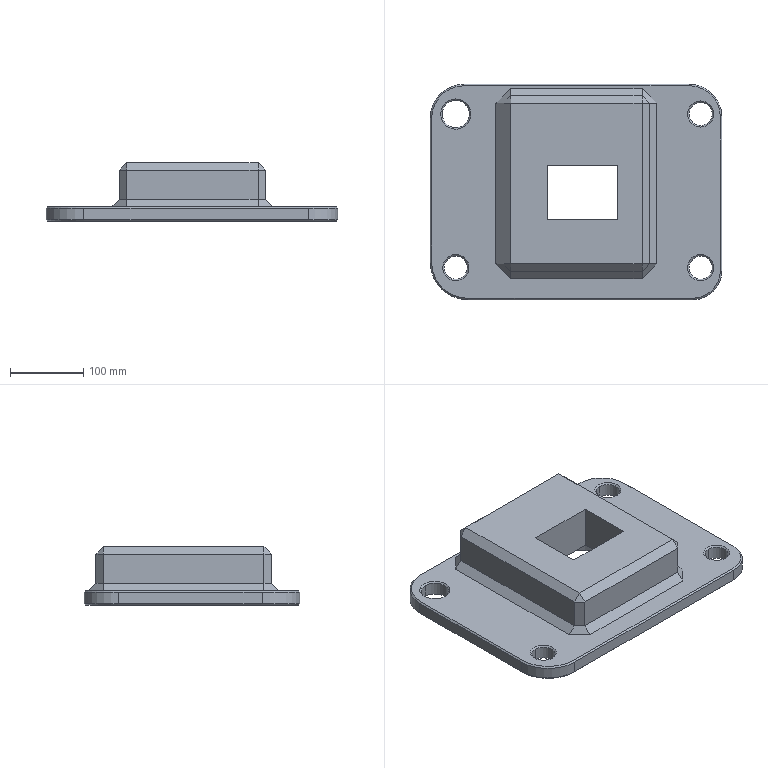Component | SolidWorks | PressurePlate-1 | 1 solid | 74 faces | box 399.22 x 295 x 80 mm | volume 4340570 mm3 | plane 44 | cone 16 | cylinder 14 | commonest cylinder face diameters 31.719 x6 37.423 x2 148.471 x2 79.887 x1 89.44 x1 93.338 x1 103.082 x1
build123d program:
from build123d import *

# Parameters (mm, degrees)
SKETCH1_W             = 295
SKETCH1_H             = 399.223
BOSS_EXTRUDE1_DEPTH   = 20
SKETCH2_W             = 240
SKETCH2_H             = 200
BOSS_EXTRUDE2_DEPTH   = 60
SKETCH3_W             = 74
SKETCH3_H             = 96
CUT_EXTRUDE1_DEPTH    = 267.314
SKETCH4_W             = 74.236
SKETCH4_H             = 20
M27_CLEARANCE_HOLE1_D = 31.719
M33_CLEARANCE_HOLE1_D = 37.423
CHAMFER1_SIZE         = 10
FILLET1_R             = 39.943
FILLET2_R             = 44.72
FILLET3_R             = 46.669
FILLET4_R             = 51.541
CHAMFER2_SIZE2        = 2
CHAMFER2_SIZE         = 2


with BuildPart() as part:
    # Sketch1 → Boss-Extrude1 (new body)
    with BuildSketch(Plane(origin=(0, 0, 190), x_dir=(-1, 0, 0), z_dir=(0, 0, -1))):
        with Locations((-0.5549, -6.793)):
            Rectangle(SKETCH1_W, SKETCH1_H)
    extrude(amount=-BOSS_EXTRUDE1_DEPTH)

    # Sketch2 → Boss-Extrude2 (add)
    with BuildSketch(Plane(origin=(0, 0, 190), x_dir=(-1, 0, 0), z_dir=(0, 0, -1))):
        with Locations((-12.055, -6.405)):
            Rectangle(SKETCH2_W, SKETCH2_H)
    extrude(amount=BOSS_EXTRUDE2_DEPTH)

    # Sketch3 → Cut-Extrude1 (cut, through all)
    with BuildSketch(Plane.XY.offset(210)):
        with Locations((0.05486, 1.595)):
            Rectangle(SKETCH3_W, SKETCH3_H)
    extrude(amount=-CUT_EXTRUDE1_DEPTH, mode=Mode.SUBTRACT)

    # Sketch4 → Cut-Revolve1 (revolve, cut)
    with BuildSketch(Plane(origin=(0, 2.202, 0), x_dir=(1, 0, 0), z_dir=(0, 1, 0))):
        with Locations((-34.987, -200)):
            Rectangle(SKETCH4_W, SKETCH4_H)
    revolve(axis=Axis((2.131, 2.202, 210), (0, 0, -1)), mode=Mode.SUBTRACT)

    # M27 Clearance Hole1 (through all)
    with Locations(Plane(origin=(0, 0, 190), x_dir=(-1, 0, 0), z_dir=(0, 0, -1))):
        with Locations((102.968, -171.325), (102.968, 163.809), (-107.267, 163.809)):
            Hole(M27_CLEARANCE_HOLE1_D / 2)

    # M33 Clearance Hole1 (through all)
    with Locations(Plane(origin=(0, 0, 190), x_dir=(-1, 0, 0), z_dir=(0, 0, -1))):
        with Locations((-107.267, -171.325)):
            Hole(M33_CLEARANCE_HOLE1_D / 2)

    # Chamfer1
    chamfer1_edges = [part.edges().sort_by_distance(p)[0] for p in [
        (132.055, -6.405, 190),
        (132.055, 93.595, 160),
        (12.055, -106.405, 190),
        (132.055, -106.405, 160),
        (-107.945, -6.405, 190),
        (-107.945, -106.405, 160),
        (12.055, 93.595, 190),
        (-107.945, 93.595, 160),
        (132.055, -6.405, 130),
        (12.055, -106.405, 130),
        (-107.945, -6.405, 130),
        (12.055, 93.595, 130),
    ]]
    chamfer(chamfer1_edges, length=CHAMFER1_SIZE)

    # Fillet1
    fillet1_edges = [part.edges().sort_by_distance(p)[0] for p in [
        (-146.945, 192.819, 200),
    ]]
    fillet(fillet1_edges, radius=FILLET1_R)

    # Fillet2
    fillet2_edges = [part.edges().sort_by_distance(p)[0] for p in [
        (148.055, 192.819, 200),
    ]]
    fillet(fillet2_edges, radius=FILLET2_R)

    # Fillet3
    fillet3_edges = [part.edges().sort_by_distance(p)[0] for p in [
        (148.055, -206.405, 200),
    ]]
    fillet(fillet3_edges, radius=FILLET3_R)

    # Fillet4
    fillet4_edges = [part.edges().sort_by_distance(p)[0] for p in [
        (-146.945, -206.405, 200),
    ]]
    fillet(fillet4_edges, radius=FILLET4_R)

    # Chamfer2
    chamfer2_edges = [part.edges().sort_by_distance(p)[0] for p in [
        (-1.833, 192.819, 190),
        (-135.246, 181.12, 190),
        (-1.833, 192.819, 210),
        (-135.246, 181.12, 210),
        (148.055, -5.818, 190),
        (134.957, 179.721, 190),
        (148.055, -5.818, 210),
        (134.957, 179.721, 210),
        (2.991, -206.405, 190),
        (134.386, -192.736, 190),
        (2.991, -206.405, 210),
        (134.386, -192.736, 210),
        (-146.945, -0.994, 190),
        (-131.849, -191.309, 190),
        (-146.945, -0.994, 210),
        (-131.849, -191.309, 210),
        (91.408, 163.809, 190),
        (-118.827, 163.809, 190),
        (-118.827, -171.325, 190),
        (88.556, -171.325, 190),
    ]]
    chamfer(chamfer2_edges, length=CHAMFER2_SIZE, length2=CHAMFER2_SIZE2)


solid = part.part

# Placed as in the assembly
solid = solid.moved(Location((-502.332, 847.548, 384.663), (180, 0, -90)))